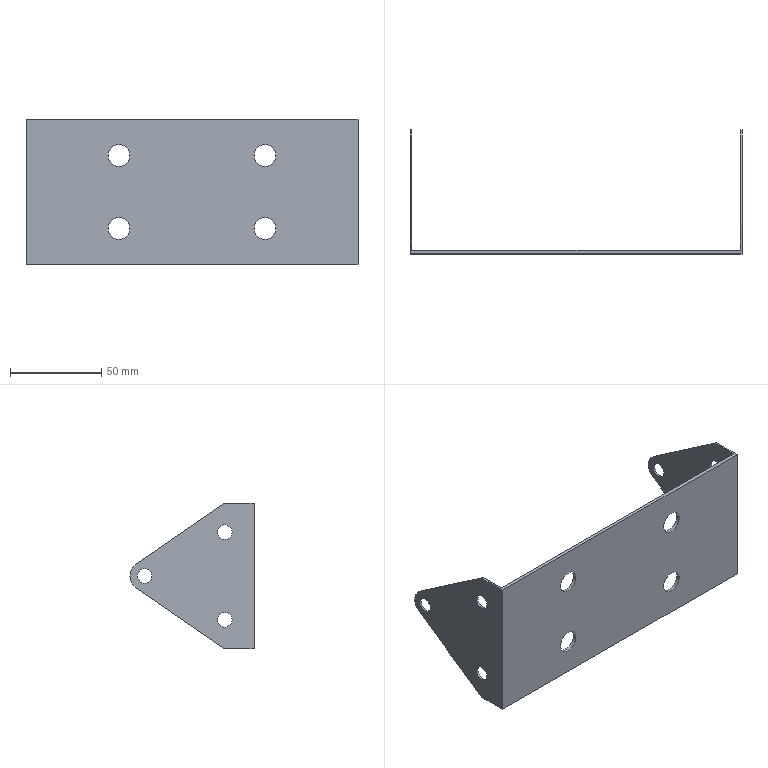Component | SolidWorks | CleaningRobotAssembly-1_CleaningBrushFixingPlate-1 | 1 solid | 36 faces | box 182 x 68 x 80 mm | volume 34740 mm3 | cylinder 24 | plane 12 | commonest cylinder face diameters 8 x12 12 x8 16 x4
build123d program:
from build123d import *

# Parameters (mm, degrees)
BOSS_EXTRUDE2_DEPTH = 80
CUT_EXTRUDE1_DEPTH  = 235
SKETCH5_R           = 4
CUT_EXTRUDE2_DEPTH  = 192
SKETCH6_R           = 6
CUT_EXTRUDE3_DEPTH  = 192


with BuildPart() as part:
    # Sketch1 → Boss-Extrude2 (new body)
    with BuildSketch(Plane.XY):
        Polygon((-90, 0), (90, 0), (90, 90), (91, 90), (91, -2), (-91, -2), (-91, 90), (-90, 90), align=None)
    extrude(amount=BOSS_EXTRUDE2_DEPTH)

    # Sketch4 → Cut-Extrude1 (cut)
    with BuildSketch(Plane(origin=(91, 0, 0), x_dir=(0, 0, -1), z_dir=(1, 0, 0))):
        with BuildLine():
            ThreePointArc((-46.678, 62.406), (-43.792, 65.044), (-40, 66))
            Line((-40, 66), (-40, 90))
            Line((-40, 90), (-80, 90))
            Line((-80, 90), (-80, 14))
            Line((-80, 14), (-46.678, 62.406))
        make_face()
        with BuildLine():
            Line((-40, 90), (-40, 66))
            ThreePointArc((-40, 66), (-36.208, 65.044), (-33.322, 62.406))
            Line((-33.322, 62.406), (0, 14))
            Line((0, 14), (0, 90))
            Line((0, 90), (-40, 90))
        make_face()
    extrude(amount=-CUT_EXTRUDE1_DEPTH, mode=Mode.SUBTRACT)

    # Sketch5 → Cut-Extrude2 (cut)
    with BuildSketch(Plane(origin=(91, 0, 0), x_dir=(0, 0, -1), z_dir=(1, 0, 0))):
        with Locations(Location((-40, 58, 0), (0, 0, 90))):
            Circle(SKETCH5_R)
        with Locations(Location((-64, 14, 0), (0, 0, 90))):
            Circle(SKETCH5_R)
        with Locations(Location((-16, 14, 0), (0, 0, 90))):
            Circle(SKETCH5_R)
    extrude(amount=-CUT_EXTRUDE2_DEPTH, mode=Mode.SUBTRACT)

    # Sketch6 → Cut-Extrude3 (cut)
    with BuildSketch(Plane(origin=(0, -2, 0), x_dir=(-1, 0, 0), z_dir=(0, -1, 0))):
        with Locations(Location((-40, -20, 0), (0, 0, 90))):
            Circle(SKETCH6_R)
        with Locations(Location((40, -20, 0), (0, 0, 90))):
            Circle(SKETCH6_R)
        with Locations(Location((-40, -60, 0), (0, 0, 90))):
            Circle(SKETCH6_R)
        with Locations(Location((40, -60, 0), (0, 0, 90))):
            Circle(SKETCH6_R)
    extrude(amount=-CUT_EXTRUDE3_DEPTH, mode=Mode.SUBTRACT)


solid = part.part

# Placed as in the assembly
solid = solid.moved(Location((310.629, -55.9, 188), (0, 0, 0)))